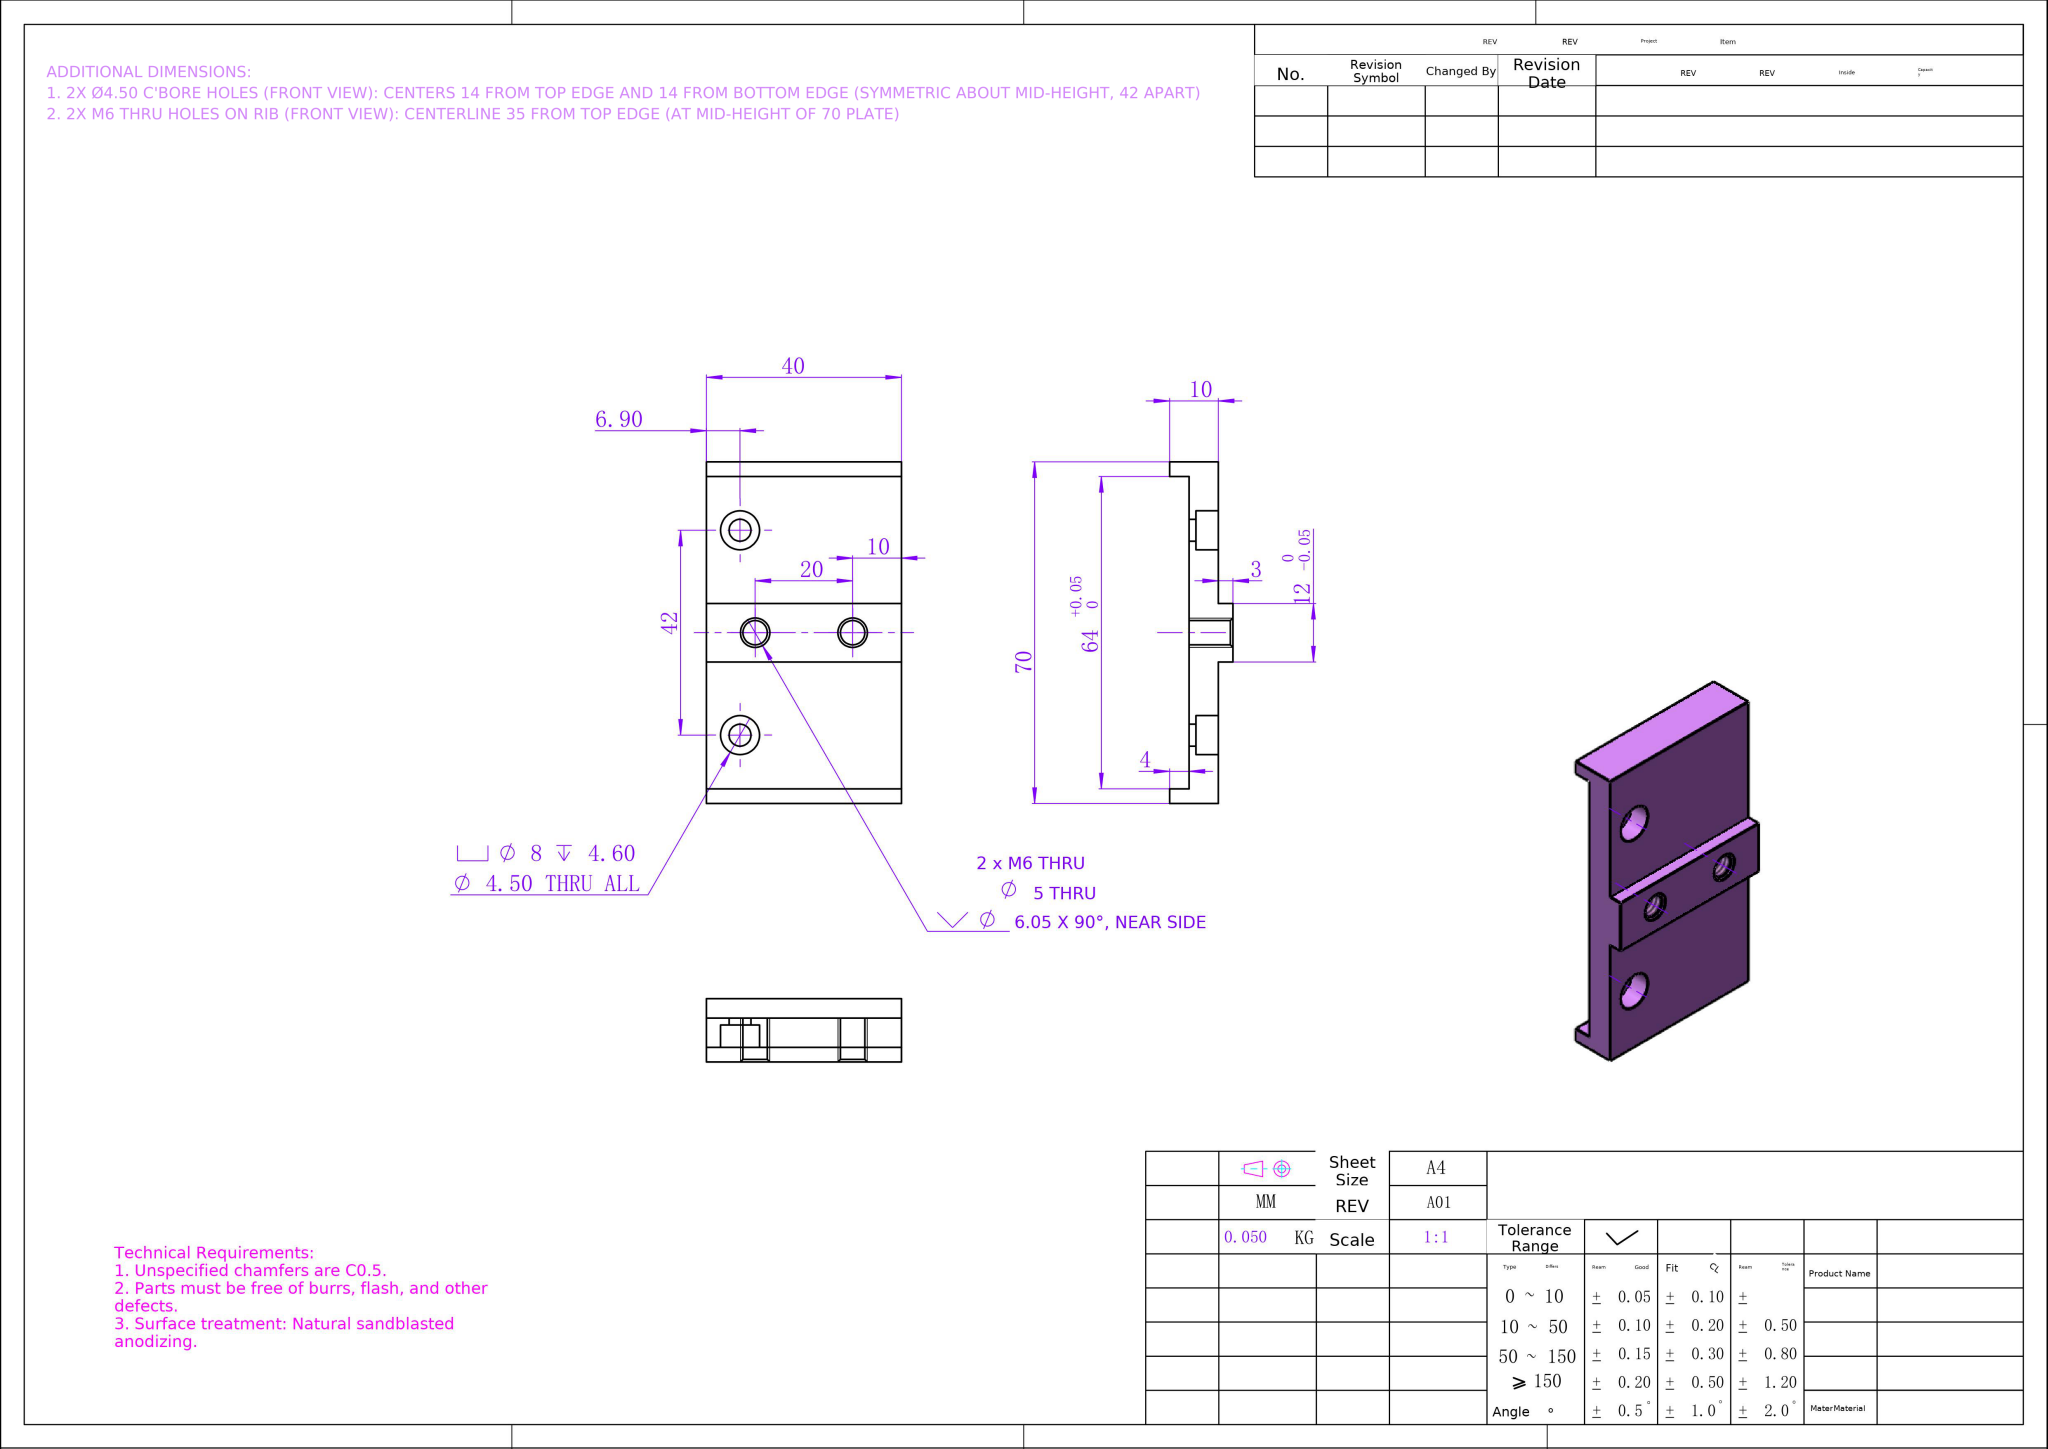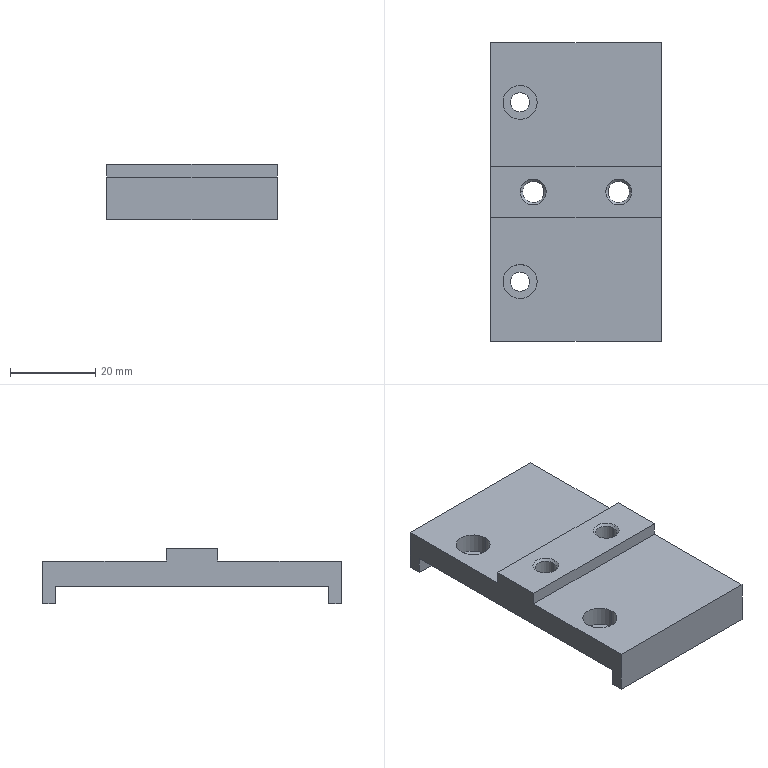Part | NX | mm | 1 solid | 32 faces | box 40 x 70 x 13 mm | volume 18335 mm3 | plane 16 | cylinder 12 | cone 4 | commonest cylinder face diameters 5 x4 4.5 x4 8 x4